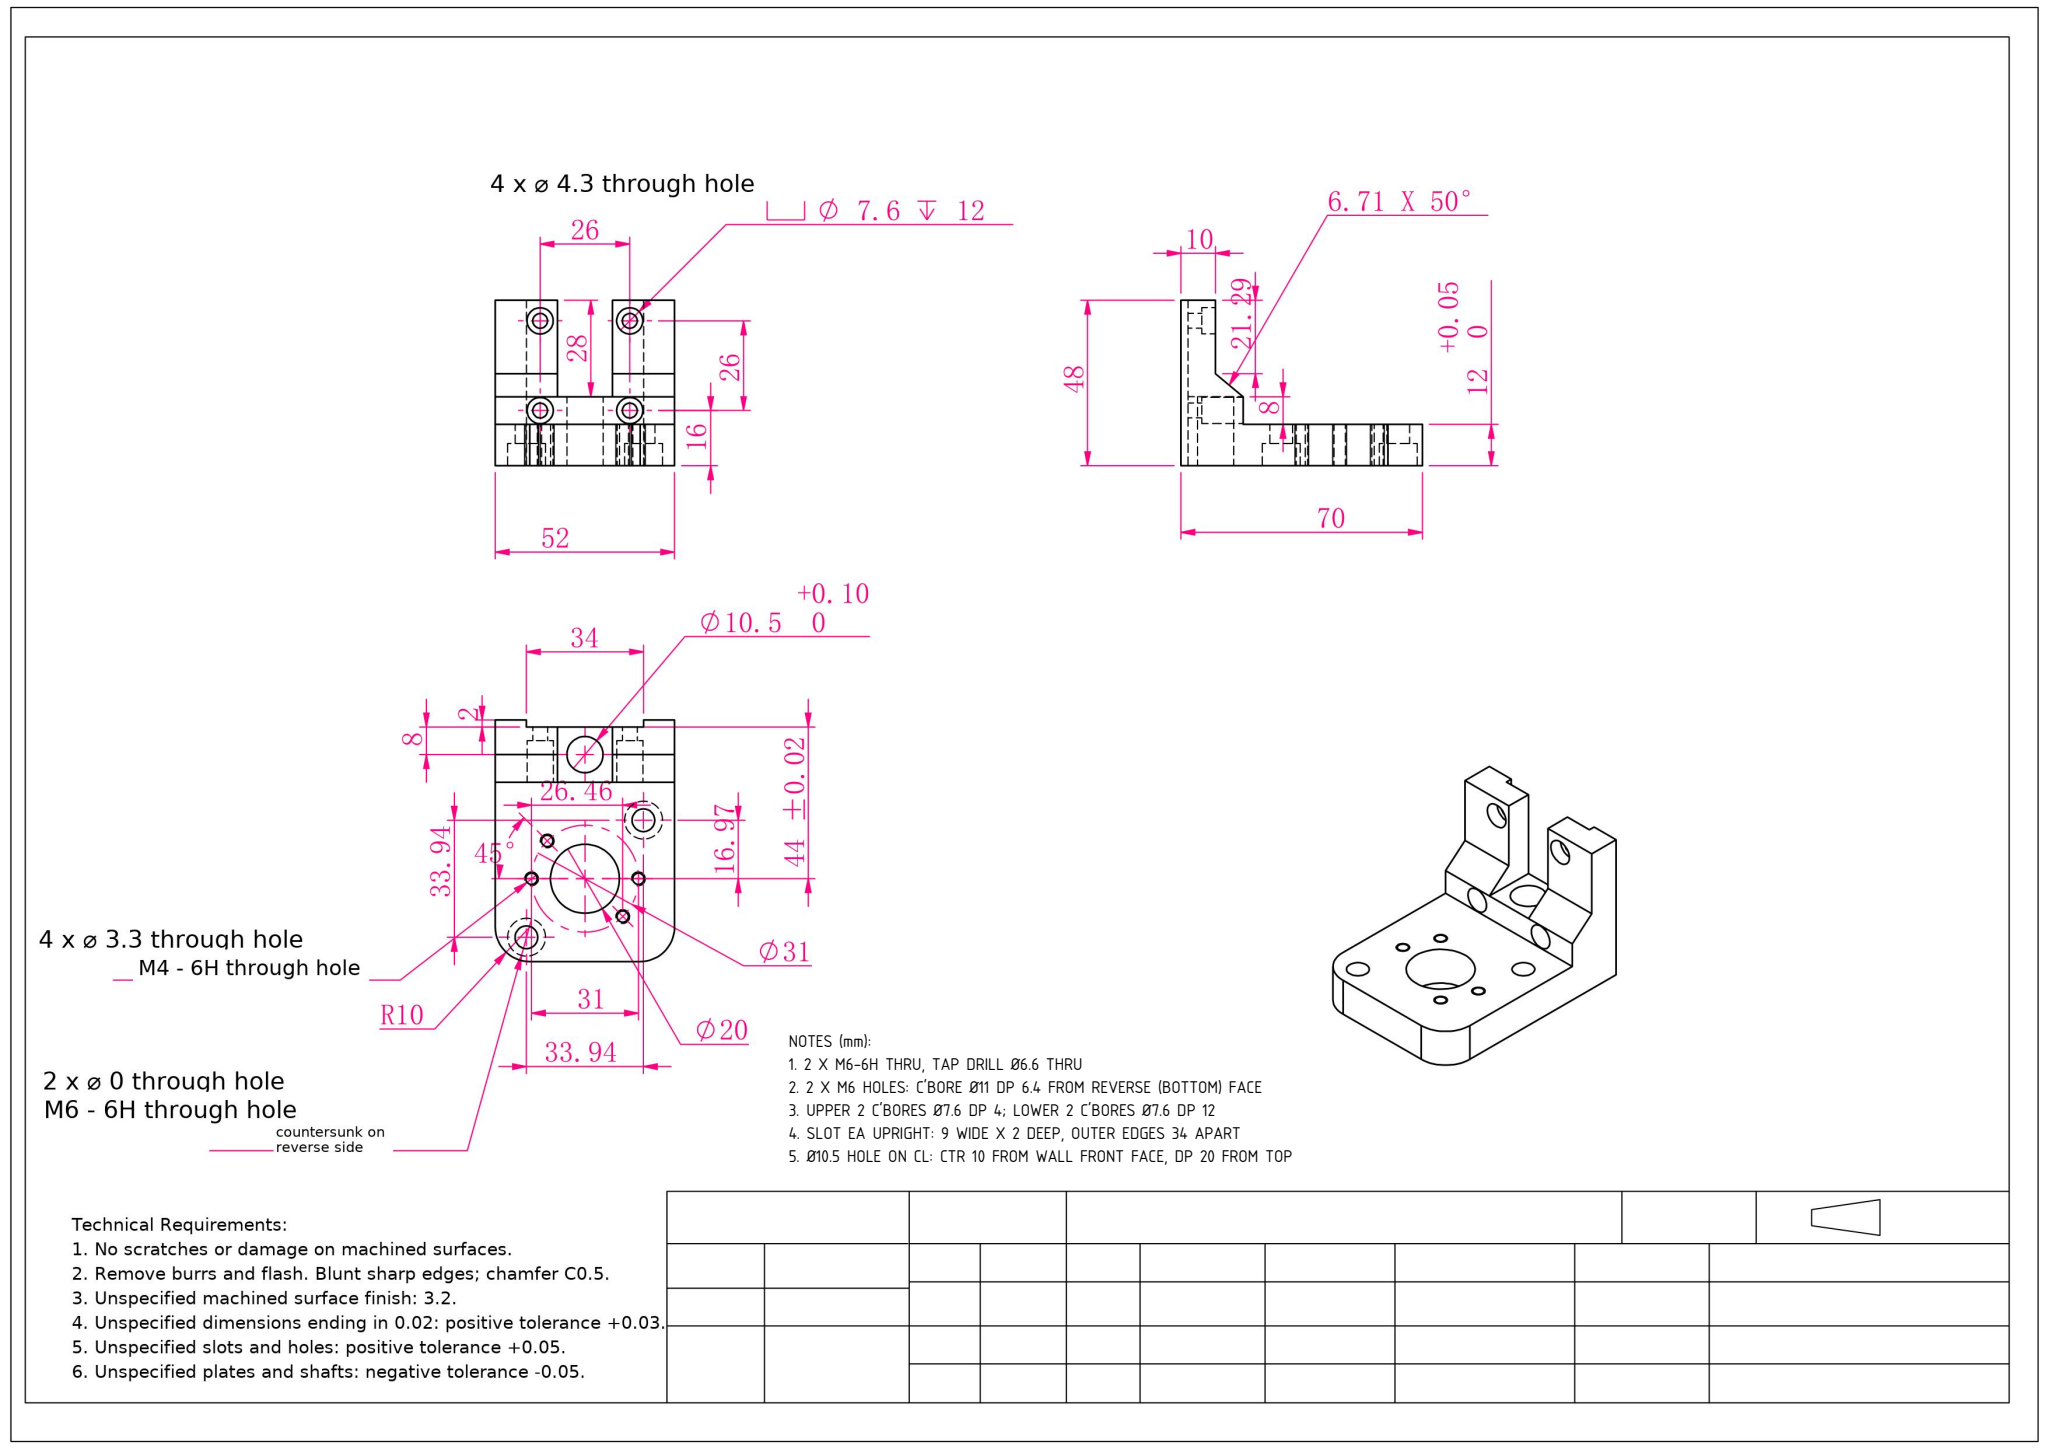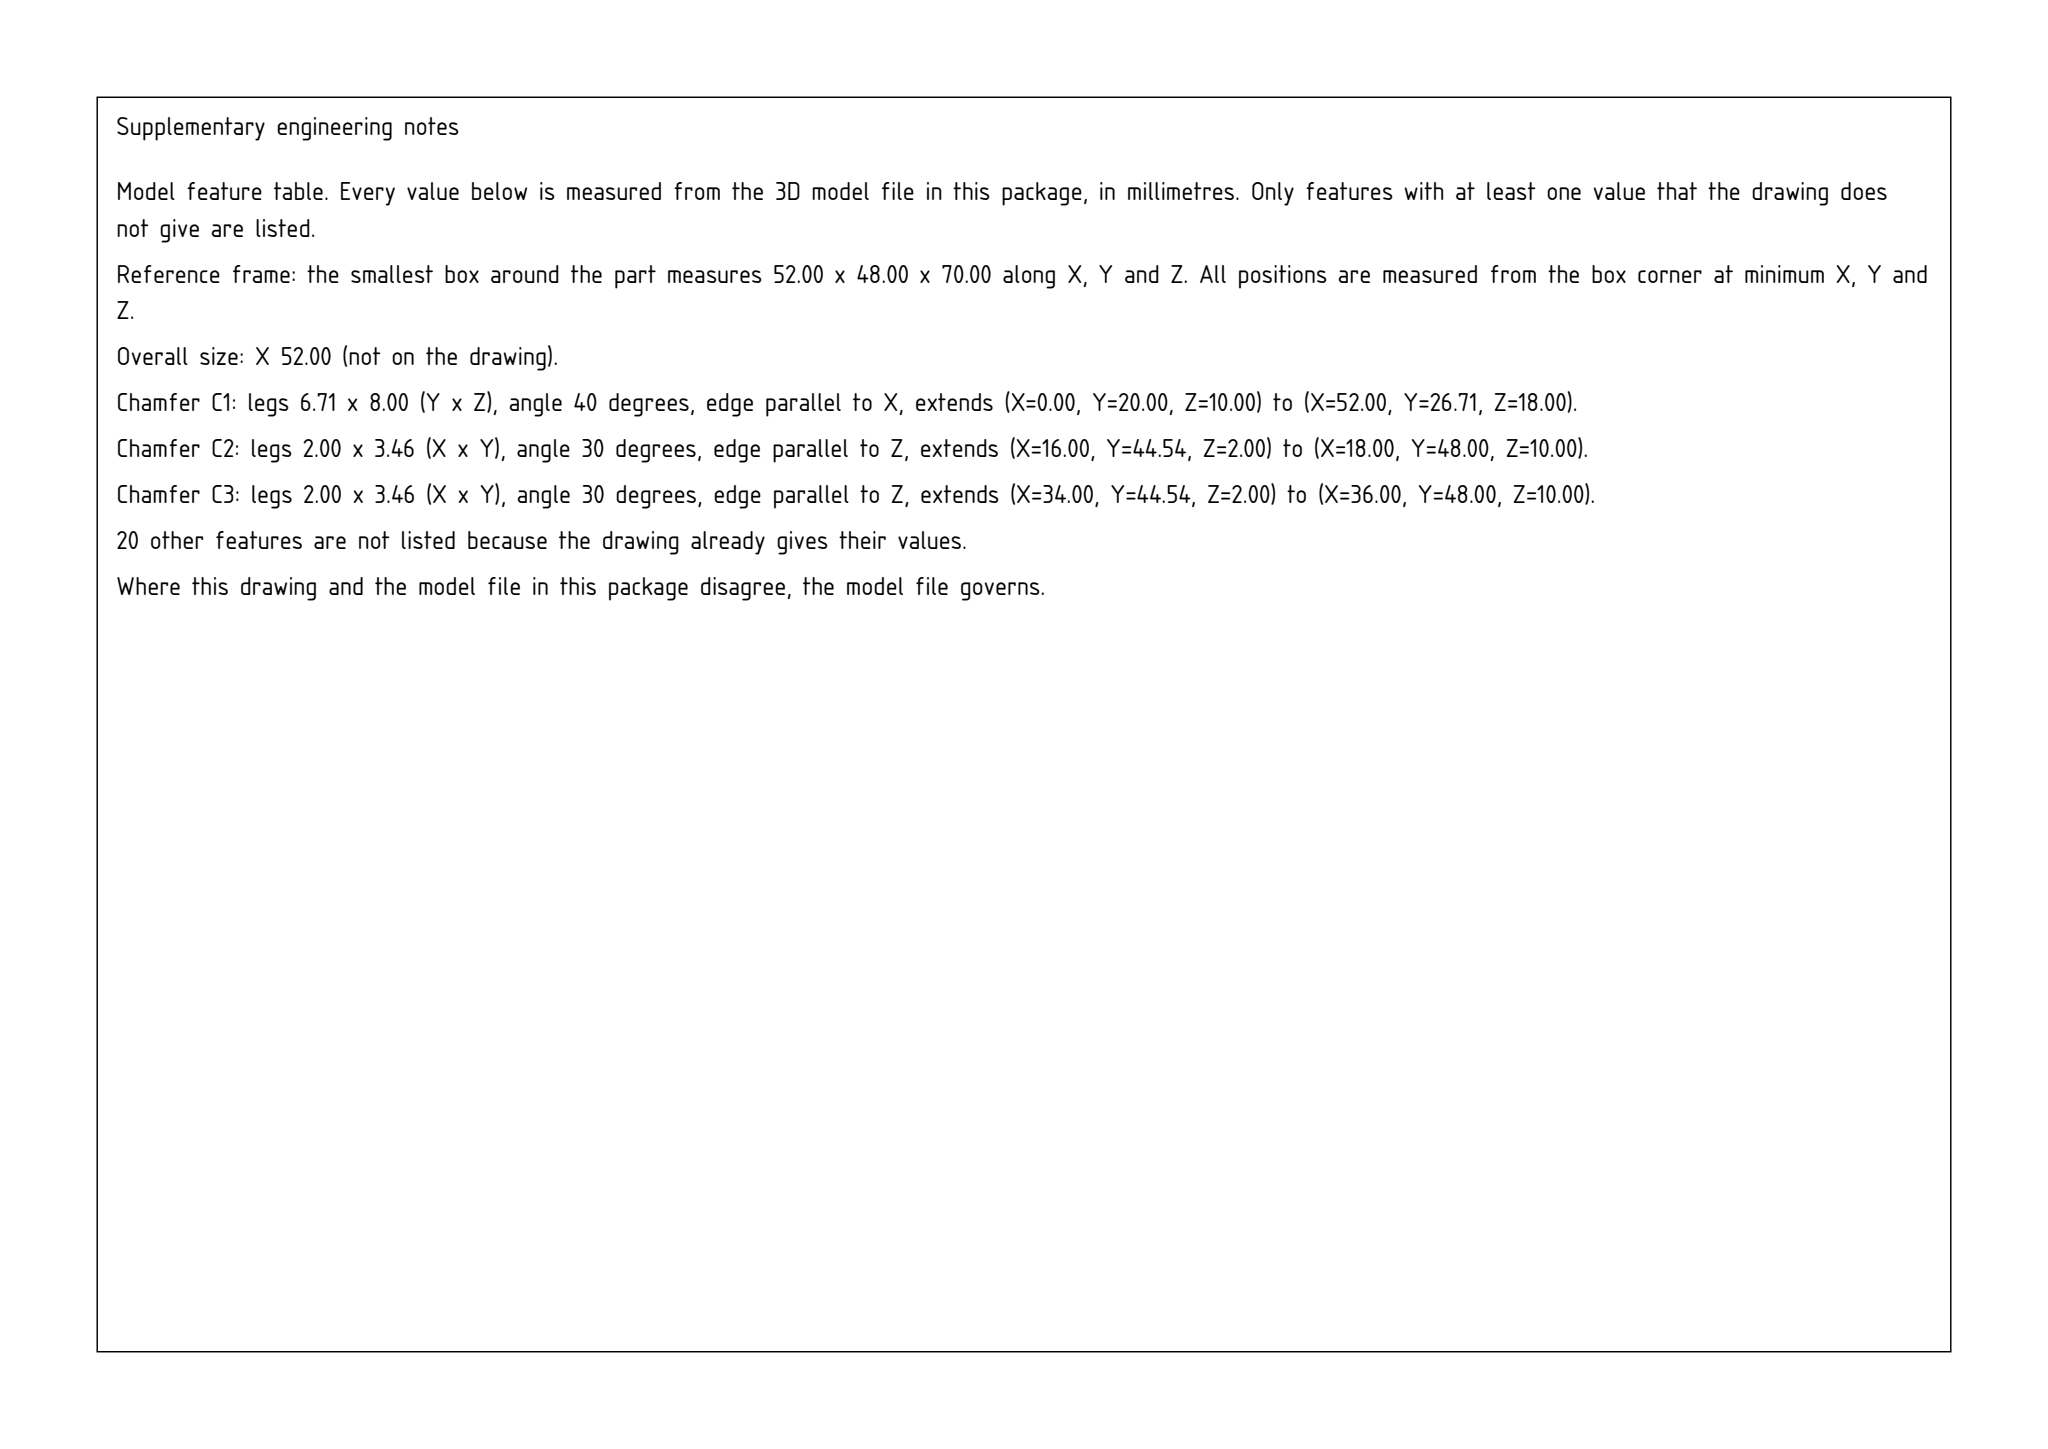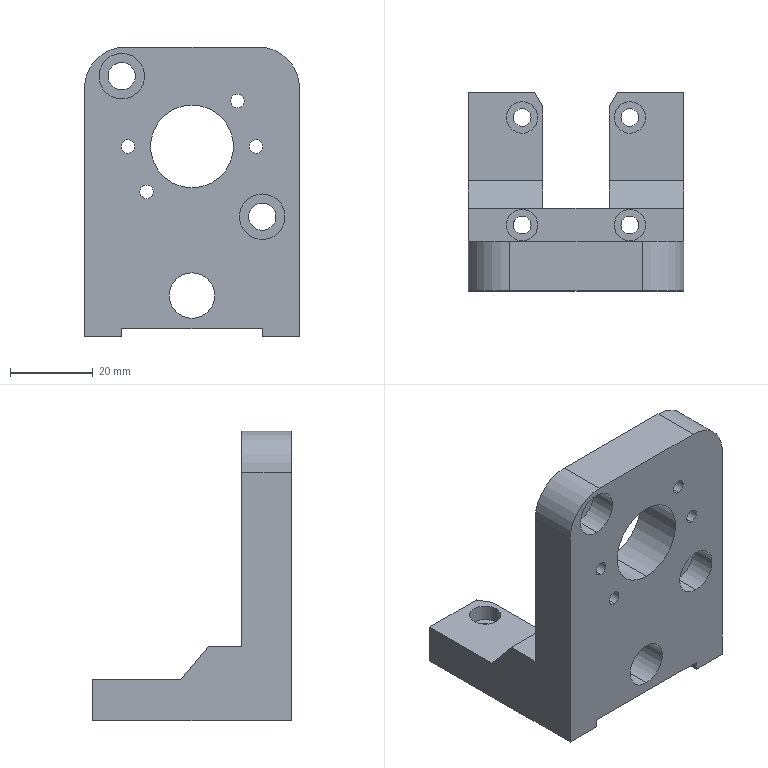Part | SolidWorks | mm | 1 solid | 66 faces | box 52 x 48 x 70 mm | volume 49911 mm3 | cylinder 38 | plane 28 | commonest cylinder face diameters 3.3 x8 7.6 x8 4.3 x8 11 x6 6.6 x4 20 x4
Drawing notes:
2 X M6-6H THRU, TAP DRILL Ø6.6 THRU | from the solid: Ø6.6 y-axis cyls at (9.03,62.97) & (42.97,29.03), len 5.6, thru 12 plate with Ø11 c'bore
2 X M6 HOLES: C'BORE Ø11 DP 6.4 FROM REVERSE (BOTTOM) FACE | from the solid: Ø11.0 y-axis cyls at (9.03,62.97) & (42.97,29.03), length 6.4, base plate y 0-12
UPPER 2 C'BORES Ø7.6 DP 4; LOWER 2 C'BORES Ø7.6 DP 12 | from the solid: Ø7.6 z-axis: (13,42)&(39,42) len 4.0; (13,16)&(39,16) len 12.0
SLOT EA UPRIGHT: 9 WIDE X 2 DEEP, OUTER EDGES 34 APART | from the solid: x planes 9 & 43 (34 apart) within uprights x0-18 & x34-52; z plane 2.0 = slot floor from z=0 face
Ø10.5 HOLE ON CL: CTR 10 FROM WALL FRONT FACE, DP 20 FROM TOP | from the solid: Ø11.0 y-axis cyl at x=26 (CL of 52), z=10 (wall 10 thk), length 20 from y=48 top face
build123d program:
from build123d import *
from OCP.BRepFilletAPI import BRepFilletAPI_MakeChamfer

# Parameters (mm, degrees)
SKETCH1_W                                       = 52
SKETCH1_H                                       = 60
EXTRUDE1_DEPTH                                  = 18
SKETCH2_W                                       = 34
SKETCH2_H                                       = 60
EXTRUDE2_DEPTH                                  = 2
M4_HEX_SOCKET_HEAD_CAP_SCREW_CBORE1_D           = 4.3
M4_HEX_SOCKET_HEAD_CAP_SCREW_CBORE1_CBORE_D     = 7.6
M4_HEX_SOCKET_HEAD_CAP_SCREW_CBORE1_CBORE_DEPTH = 12
SKETCH26_R                                      = 5.5
CUT_EXTRUDE4_DEPTH                              = 82.413
SKETCH28_W                                      = 16
SKETCH28_H                                      = 16
CUT_EXTRUDE5_DEPTH                              = 40
SKETCH29_W                                      = 52
SKETCH29_H                                      = 12
BOSS_EXTRUDE1_DEPTH                             = 52
SKETCH30_R                                      = 10
CUT_EXTRUDE6_DEPTH                              = 40
FILLET1_R                                       = 10
M6_HEX_SOCKET_HEAD_CAP_SCREW_CBORE1_D           = 6.6
M6_HEX_SOCKET_HEAD_CAP_SCREW_CBORE1_CBORE_D     = 11
M6_HEX_SOCKET_HEAD_CAP_SCREW_CBORE1_CBORE_DEPTH = 6.4
M4_TAPPED_HOLE1_D                               = 3.3
SKETCH35_W                                      = 52
SKETCH35_H                                      = 12
CUT_EXTRUDE7_DEPTH                              = 95.91
CUT_EXTRUDE8_DEPTH                              = 100.539
CUT_EXTRUDE8_DEPTH_BACK                         = 100.539
CHAMFER1_SIZE                                   = 2
CHAMFER1_SIZE2                                  = 3.464


with BuildPart() as part:
    # Sketch1 → Extrude1 (new body)
    with BuildSketch(Plane.XY):
        with Locations((26, 30)):
            Rectangle(SKETCH1_W, SKETCH1_H)
    extrude(amount=EXTRUDE1_DEPTH)

    # Sketch2 → Extrude2 (cut)
    with BuildSketch(Plane(origin=(0, 0, 0), x_dir=(-1, 0, 0), z_dir=(0, 0, -1))):
        with Locations((-26, 30)):
            Rectangle(SKETCH2_W, SKETCH2_H)
    extrude(amount=-EXTRUDE2_DEPTH, mode=Mode.SUBTRACT)

    # M4 Hex Socket Head Cap Screw CBORE1 (through all)
    with Locations(Plane.XY.offset(18)):
        with Locations((13, 16), (13, 42), (39, 42), (39, 16)):
            CounterBoreHole(M4_HEX_SOCKET_HEAD_CAP_SCREW_CBORE1_D / 2, M4_HEX_SOCKET_HEAD_CAP_SCREW_CBORE1_CBORE_D / 2, M4_HEX_SOCKET_HEAD_CAP_SCREW_CBORE1_CBORE_DEPTH)

    # Sketch26 → Cut-Extrude4 (cut, through all)
    with BuildSketch(Plane(origin=(0, 60, 0), x_dir=(1, 0, 0), z_dir=(0, 1, 0))):
        with Locations(Location((26, -10, 0), (0, 0, 270))):
            Circle(SKETCH26_R)
    extrude(amount=-CUT_EXTRUDE4_DEPTH, mode=Mode.SUBTRACT)

    # Sketch28 → Cut-Extrude5 (cut)
    with BuildSketch(Plane(origin=(0, 60, 0), x_dir=(1, 0, 0), z_dir=(0, 1, 0))):
        with Locations((26, -10)):
            Rectangle(SKETCH28_W, SKETCH28_H)
    extrude(amount=-CUT_EXTRUDE5_DEPTH, mode=Mode.SUBTRACT)

    # Sketch29 → Boss-Extrude1 (add)
    with BuildSketch(Plane.XY.offset(18)):
        with Locations((26, 6)):
            Rectangle(SKETCH29_W, SKETCH29_H)
    extrude(amount=BOSS_EXTRUDE1_DEPTH)

    # Sketch30 → Cut-Extrude6 (cut)
    with BuildSketch(Plane.XZ):
        with Locations(Location((26, 46, 0), (0, 0, 270))):
            Circle(SKETCH30_R)
    extrude(amount=-CUT_EXTRUDE6_DEPTH, mode=Mode.SUBTRACT)

    # Fillet1
    fillet1_edges = [part.edges().sort_by_distance(p)[0] for p in [
        (0, 6, 70),
        (52, 6, 70),
    ]]
    fillet(fillet1_edges, radius=FILLET1_R)

    # M6 Hex Socket Head Cap Screw CBORE1 (through all)
    with Locations(Plane(origin=(0, 0, 0), x_dir=(-1, 0, 0), z_dir=(0, -1, 0))):
        with Locations((-9.029, -62.971), (-42.971, -29.029)):
            CounterBoreHole(M6_HEX_SOCKET_HEAD_CAP_SCREW_CBORE1_D / 2, M6_HEX_SOCKET_HEAD_CAP_SCREW_CBORE1_CBORE_D / 2, M6_HEX_SOCKET_HEAD_CAP_SCREW_CBORE1_CBORE_DEPTH)

    # M4 Tapped Hole1 (through all)
    with Locations(Plane(origin=(0, 12, 0), x_dir=(1, 0, 0), z_dir=(0, 1, 0))):
        with Locations((15.04, -35.04), (41.5, -46), (36.96, -56.96), (10.5, -46)):
            Hole(M4_TAPPED_HOLE1_D / 2)

    # Sketch35 → Cut-Extrude7 (cut, through all)
    with BuildSketch(Plane.XY.offset(18)):
        with Locations((26, 54)):
            Rectangle(SKETCH35_W, SKETCH35_H)
    extrude(amount=-CUT_EXTRUDE7_DEPTH, mode=Mode.SUBTRACT)

    # Sketch36 → Cut-Extrude8 (cut, two sides: drawn at the far end of the back side and taken through both)
    with BuildSketch(Plane.ZY.offset(-CUT_EXTRUDE8_DEPTH_BACK)):
        Polygon((10, 48), (10, 26.713), (18, 20), (18, 48), align=None)
    extrude(amount=CUT_EXTRUDE8_DEPTH + CUT_EXTRUDE8_DEPTH_BACK, mode=Mode.SUBTRACT)

    # Chamfer1: one chamfer whose edges measure the first distance from different faces: ONE call of the kernel's chamfer builder (chamfer() names one face for all edges)
    chamfer1_edges_1 = [part.edges().sort_by_distance(p)[0] for p in [
        (18, 48, 6),
    ]]
    chamfer1_side_1 = [part.faces().sort_by_distance(p)[0] for p in [
        (8.5, 48, 5.444),
    ]]
    chamfer1_edges_2 = [part.edges().sort_by_distance(p)[0] for p in [
        (34, 48, 6),
    ]]
    chamfer1_side_2 = [part.faces().sort_by_distance(p)[0] for p in [
        (43.5, 48, 5.444),
    ]]
    chamfer1 = BRepFilletAPI_MakeChamfer(part.part.solid().wrapped)
    for e in chamfer1_edges_1:
        chamfer1.Add(CHAMFER1_SIZE, CHAMFER1_SIZE2, e.wrapped, chamfer1_side_1[0].wrapped)  # the first distance lies on this face
    for e in chamfer1_edges_2:
        chamfer1.Add(CHAMFER1_SIZE, CHAMFER1_SIZE2, e.wrapped, chamfer1_side_2[0].wrapped)  # the first distance lies on this face
    add(Compound.cast(chamfer1.Shape()), mode=Mode.REPLACE)


solid = part.part